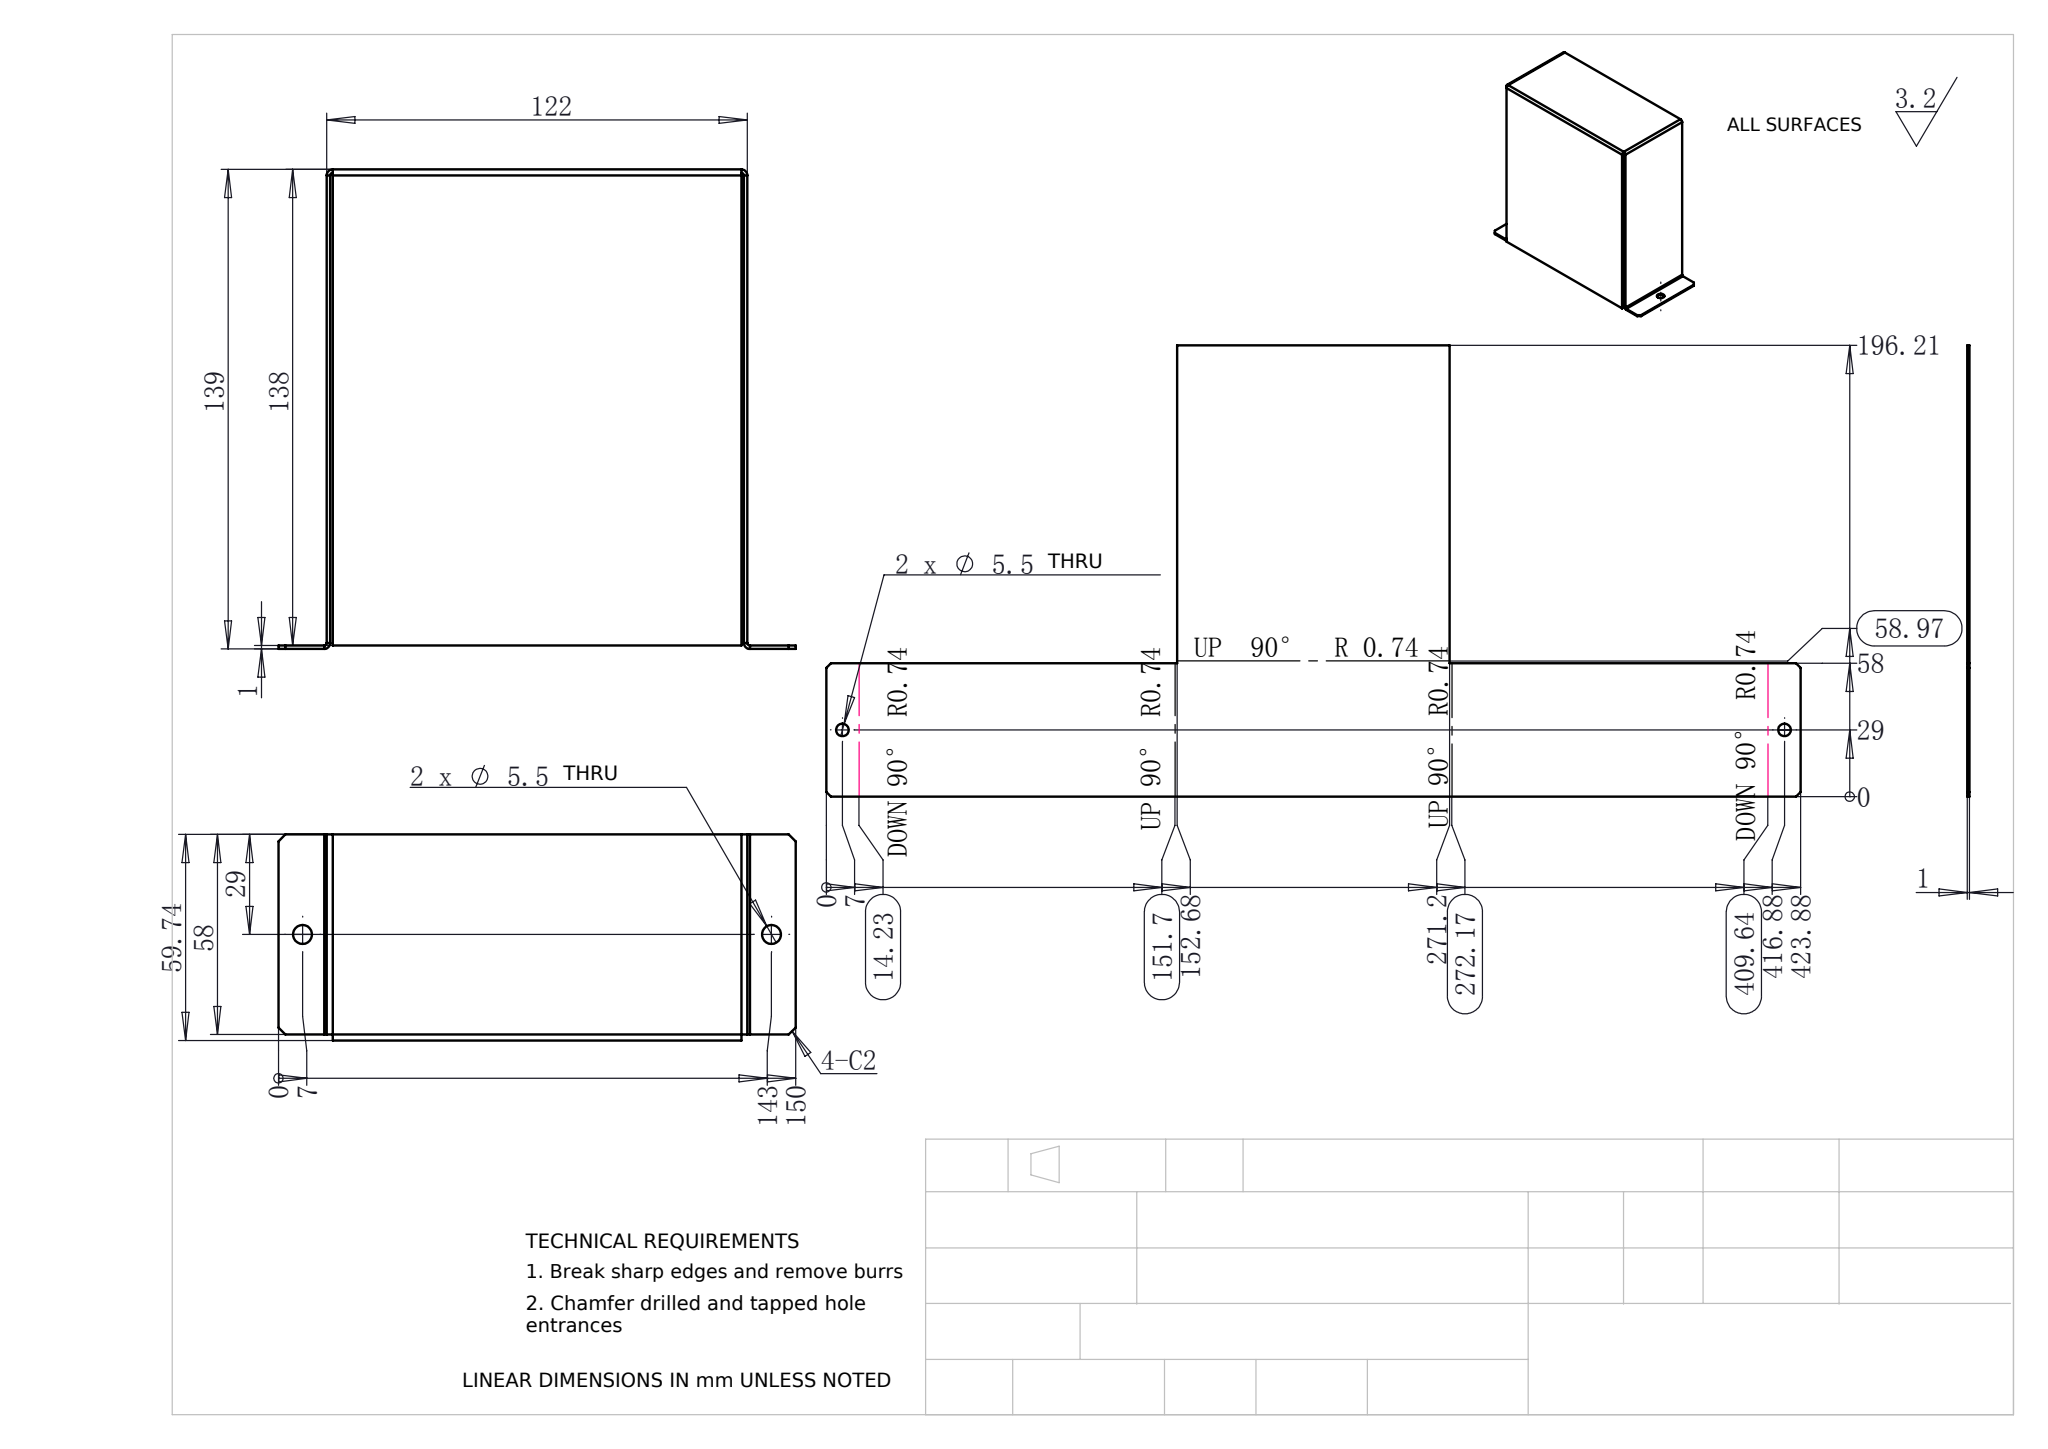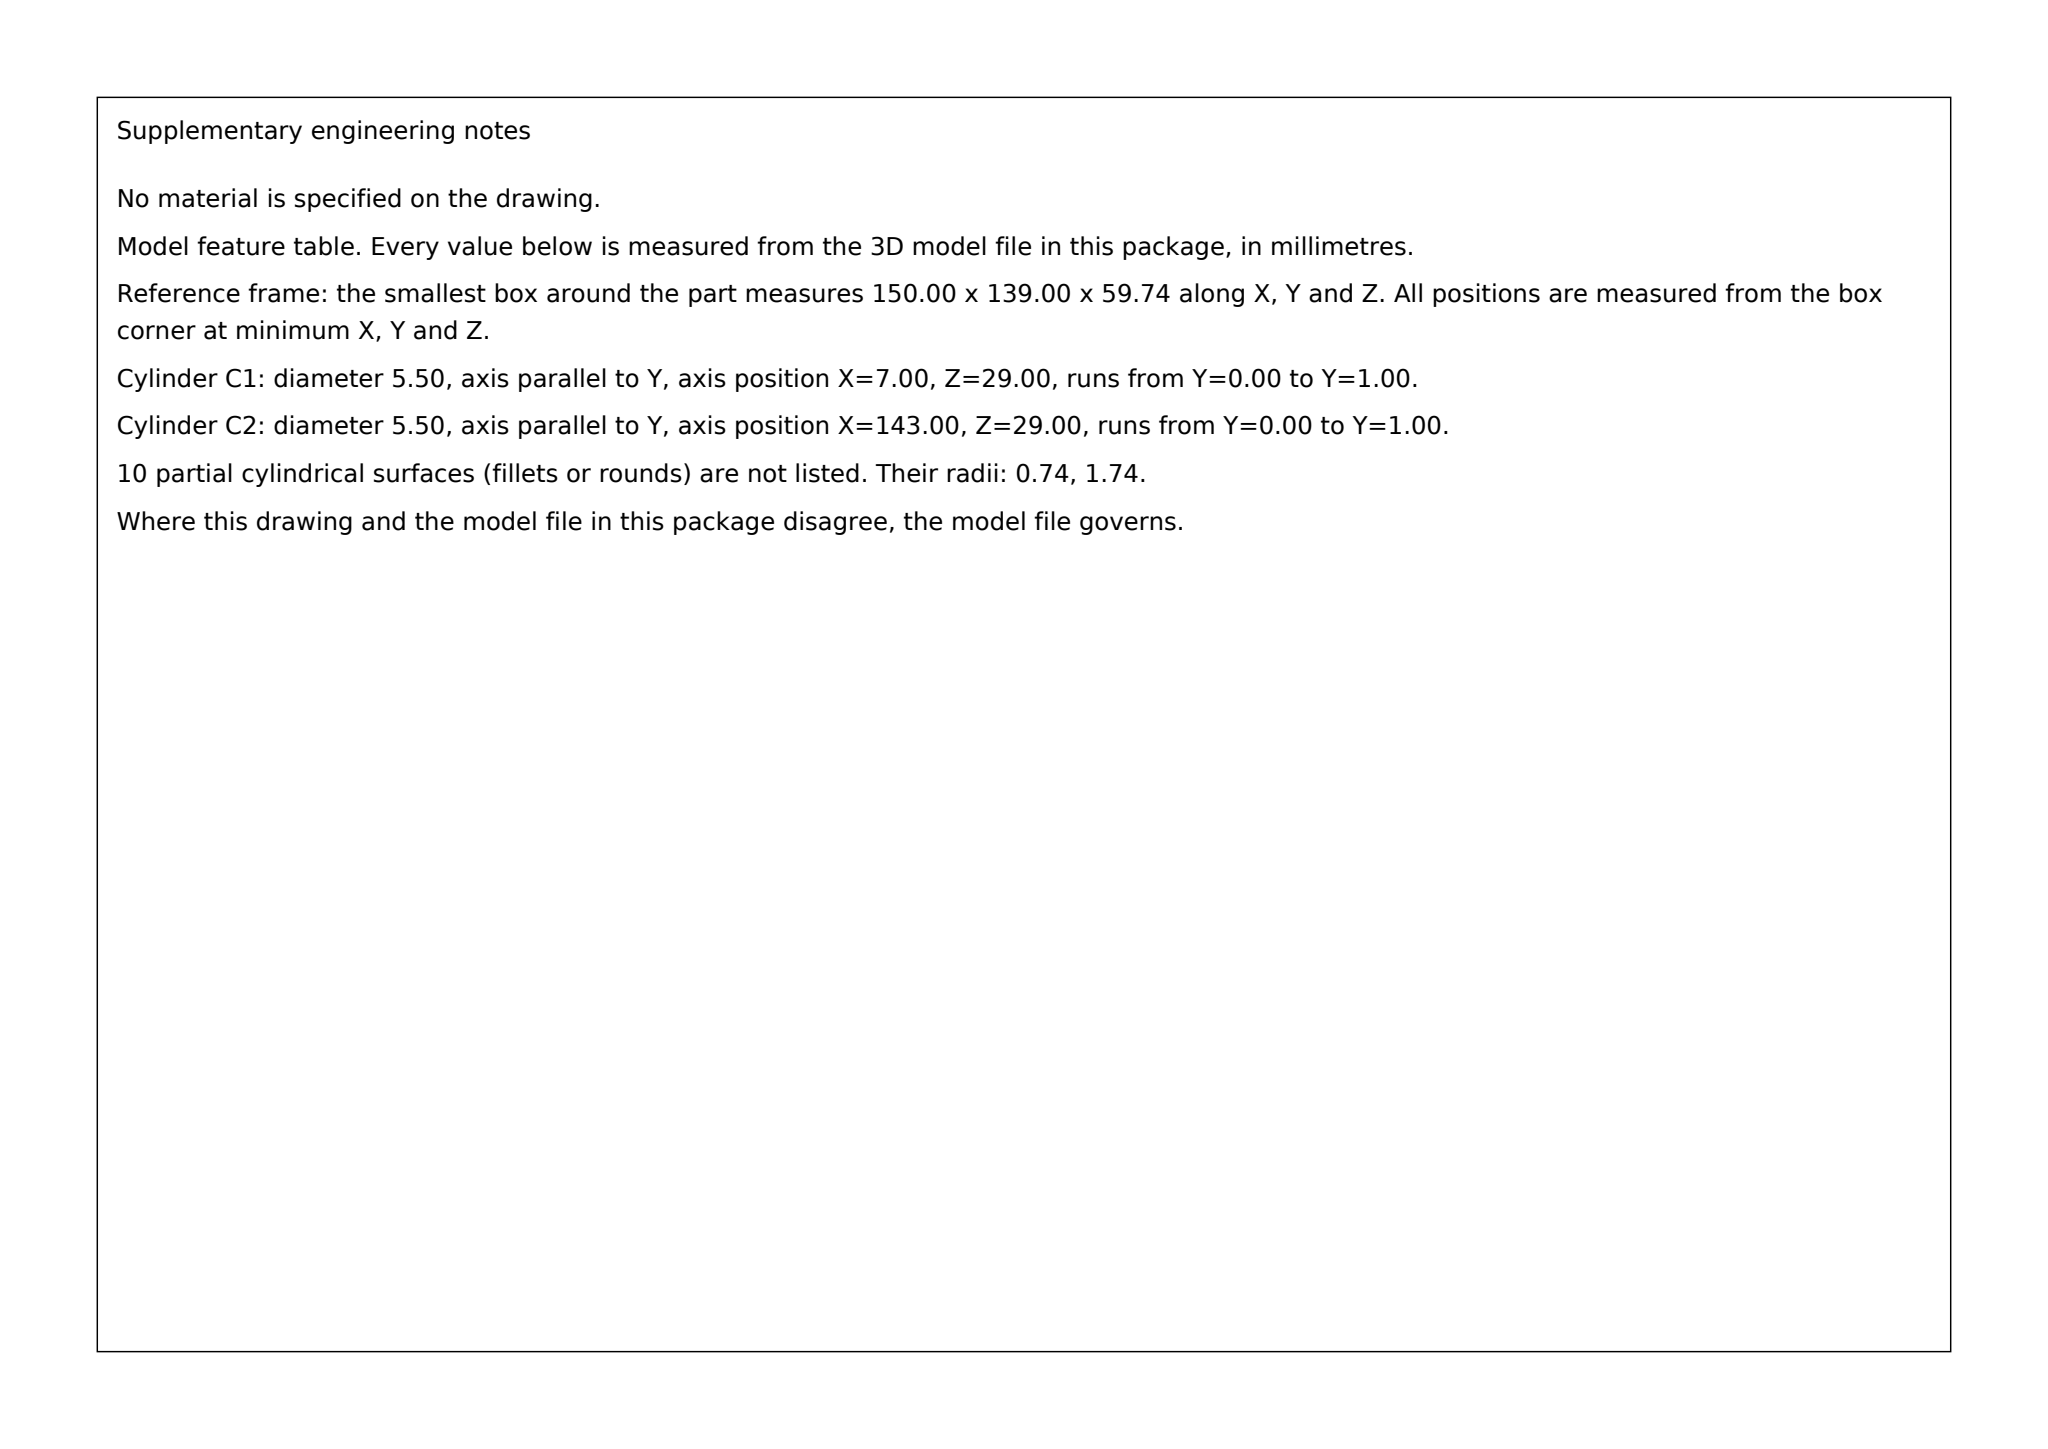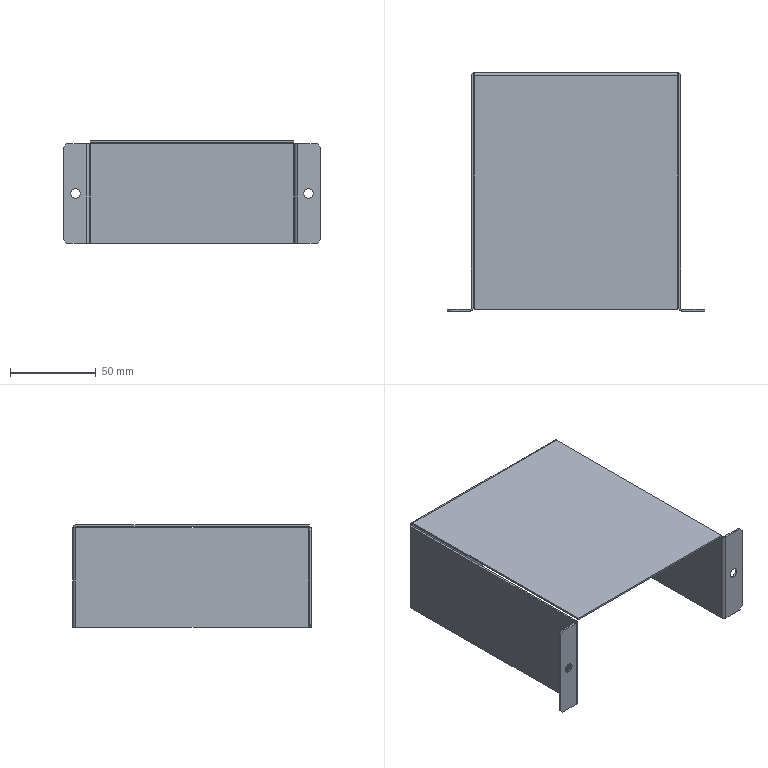Part | SolidWorks | mm | 1 solid | 54 faces | box 150 x 139 x 59.74 mm | volume 40910 mm3 | plane 40 | cylinder 14 | commonest cylinder face diameters 3.473 x5 1.473 x5 5.5 x4